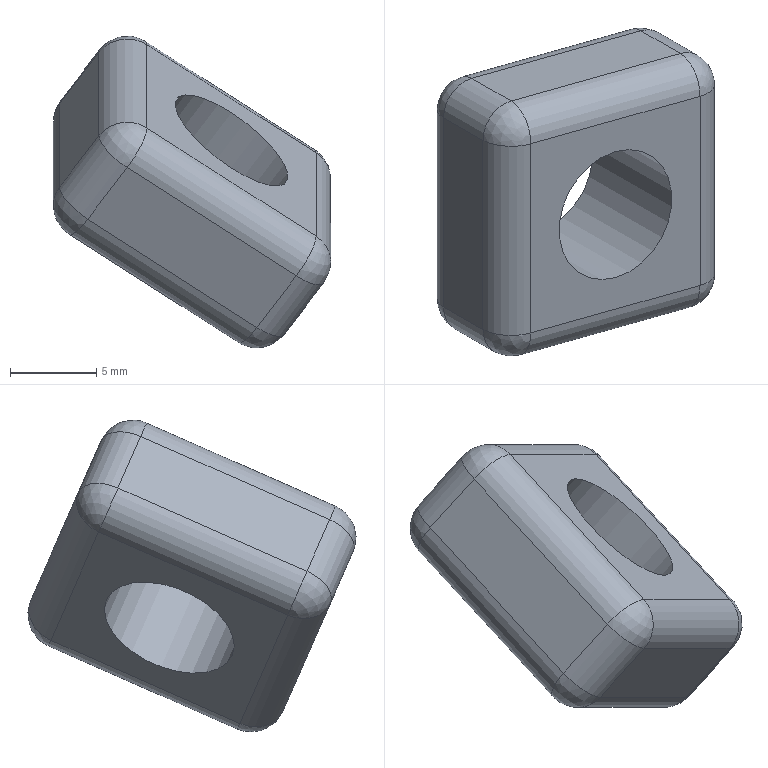Component | NX | HUA_KUAI | 1 solid | 27 faces | volume 1519 mm3 | cylinder 13 | sphere 8 | plane 6 | commonest cylinder face diameters 4 x12 8 x1